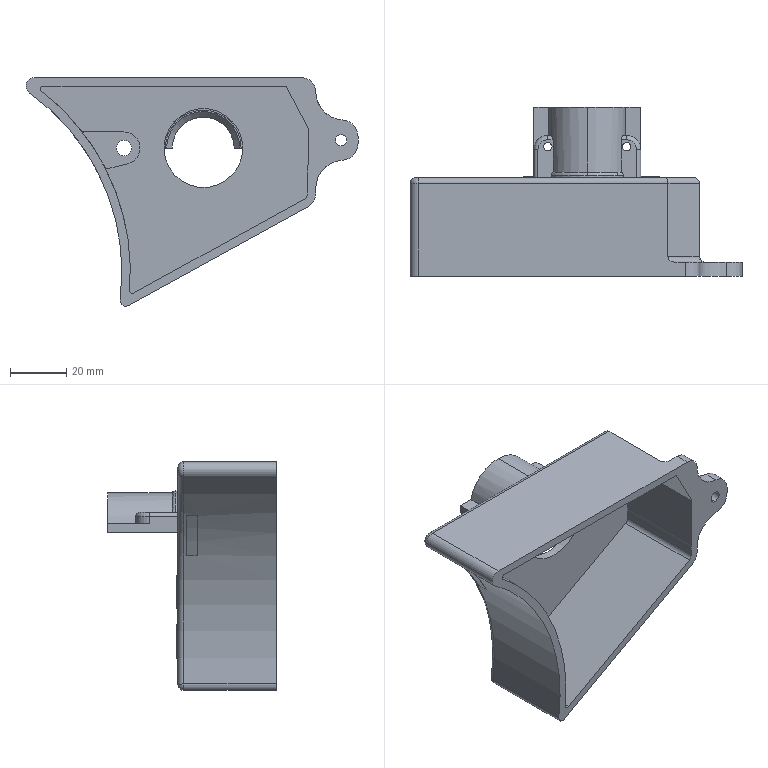Component | SolidWorks | cache ein aus-1 | 1 solid | 266 faces | box 117.88 x 60 x 81.16 mm | volume 48175 mm3 | spline 111 | cylinder 75 | plane 71 | torus 7 | cone 1 | sphere 1 | commonest cylinder face diameters 0.6 x29 4 x11 3 x8 2 x4 28 x4 10 x4 5.5 x2 20 x2